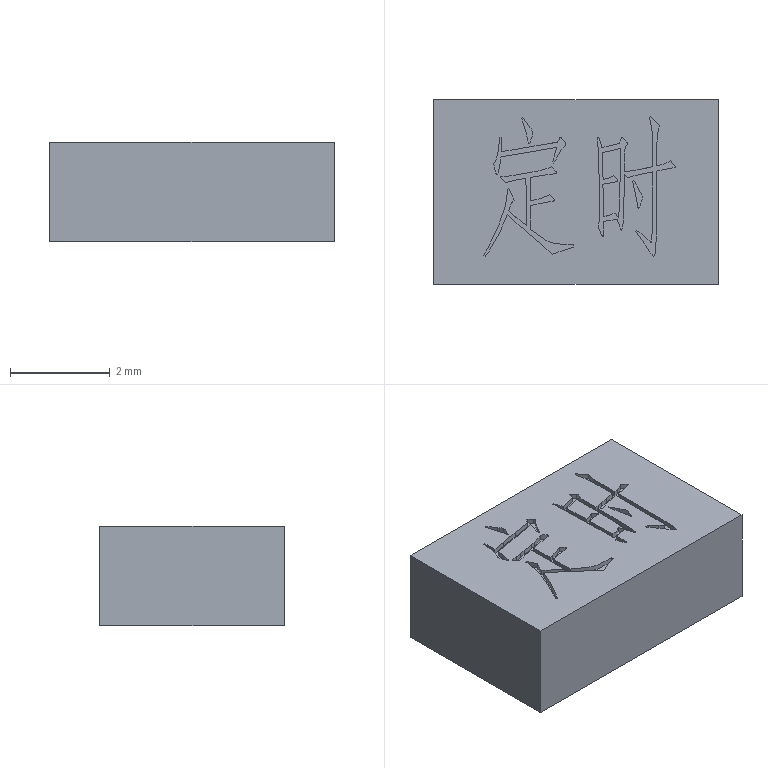Component | SolidWorks | Button3-1 | 1 solid | 162 faces | box 5.7 x 3.7 x 2 mm | volume 42 mm3 | plane 117 | spline 45
build123d program:
from build123d import *

# Parameters (mm, degrees)
SKETCH1_W           = 5.7
SKETCH1_H           = 3.7
BOSS_EXTRUDE1_DEPTH = 2
CUT_EXTRUDE1_DEPTH  = 0.1


with BuildPart() as part:
    # Sketch1 → Boss-Extrude1 (new body)
    with BuildSketch(Plane.XY):
        with Locations((2.85, 1.85)):
            Rectangle(SKETCH1_W, SKETCH1_H)
    extrude(amount=BOSS_EXTRUDE1_DEPTH)

    # Sketch2 → Cut-Extrude1 (cut)
    # profile 1 of 5: a face of its own
    with BuildSketch(Plane.XY.offset(2)):
        with BuildLine():
            Line((1.002, 0.5857), (1.037, 0.6457))
            add(Edge.make_bspline(
                [(1.037, 0.6457), (1.038, 0.6476), (1.041, 0.6531), (1.047, 0.6641), (1.055, 0.6808), (1.062, 0.6935), (1.066, 0.7007)],
                knots=[0, 0, 0, 0, 0.405, 1.215, 2.417, 4, 4, 4, 4], degree=3))
            Line((1.066, 0.7007), (1.146, 0.8473))
            add(Edge.make_bspline(
                [(1.146, 0.8473), (1.16, 0.8735), (1.189, 0.9291), (1.23, 1.019), (1.275, 1.121), (1.313, 1.211), (1.343, 1.286), (1.364, 1.341), (1.383, 1.393), (1.399, 1.442), (1.413, 1.488), (1.426, 1.531), (1.436, 1.572), (1.452, 1.647), (1.468, 1.758), (1.476, 1.856), (1.48, 1.906)],
                knots=[0, 0, 0, 0, 1.106, 2.349, 3.736, 5.256, 6.032, 6.768, 7.459, 8.107, 8.709, 9.274, 9.795, 10.281, 12.137, 14, 14, 14, 14], degree=3))
            Line((1.48, 1.906), (1.506, 1.911))
            Line((1.506, 1.911), (1.609, 1.687))
            add(Edge.make_bspline(
                [(1.609, 1.687), (1.601, 1.681), (1.587, 1.669), (1.573, 1.652), (1.566, 1.638), (1.561, 1.627), (1.554, 1.611), (1.547, 1.591), (1.537, 1.567), (1.528, 1.538), (1.515, 1.505), (1.507, 1.481), (1.503, 1.469)],
                knots=[0, 0, 0, 0, 1.223, 2.28, 2.612, 3.122, 3.811, 4.68, 5.735, 6.98, 8.395, 10, 10, 10, 10], degree=3))
            add(Edge.make_bspline(
                [(1.503, 1.469), (1.527, 1.447), (1.578, 1.401), (1.661, 1.331), (1.754, 1.255), (1.819, 1.202), (1.854, 1.175)],
                knots=[0, 0, 0, 0, 0.8497, 1.799, 2.85, 4, 4, 4, 4], degree=3))
            Line((1.854, 1.175), (1.848, 2.122))
            add(Edge.make_bspline(
                [(1.848, 2.122), (1.814, 2.116), (1.744, 2.106), (1.642, 2.086), (1.541, 2.062), (1.475, 2.042), (1.443, 2.032)],
                knots=[0, 0, 0, 0, 1.012, 2.016, 3.011, 4, 4, 4, 4], degree=3))
            Line((1.443, 2.032), (1.356, 2.122))
            add(Edge.make_bspline(
                [(1.356, 2.122), (1.352, 2.126), (1.344, 2.133), (1.339, 2.148), (1.35, 2.158), (1.359, 2.159), (1.365, 2.159)],
                knots=[0, 0, 0, 0, 1.34, 2.141, 2.818, 4, 4, 4, 4], degree=3))
            Line((1.365, 2.159), (1.474, 2.165))
            Line((1.474, 2.165), (1.612, 2.182))
            Line((1.612, 2.182), (1.739, 2.205))
            Line((1.739, 2.205), (1.989, 2.251))
            Line((1.989, 2.251), (2.084, 2.268))
            add(Edge.make_bspline(
                [(2.084, 2.268), (2.112, 2.274), (2.164, 2.284), (2.236, 2.305), (2.299, 2.328), (2.335, 2.348), (2.352, 2.358)],
                knots=[0, 0, 0, 0, 1.191, 2.249, 3.183, 4, 4, 4, 4], degree=3))
            Line((2.352, 2.358), (2.449, 2.266))
            add(Edge.make_bspline(
                [(2.449, 2.266), (2.454, 2.26), (2.462, 2.25), (2.466, 2.232), (2.455, 2.219), (2.444, 2.218), (2.438, 2.217)],
                knots=[0, 0, 0, 0, 1.282, 2.156, 2.913, 4, 4, 4, 4], degree=3))
            Line((2.438, 2.217), (2.225, 2.188))
            Line((2.225, 2.188), (1.934, 2.139))
            Line((1.934, 2.139), (1.94, 1.67))
            Line((1.94, 1.67), (2.026, 1.69))
            add(Edge.make_bspline(
                [(2.026, 1.69), (2.056, 1.697), (2.113, 1.711), (2.191, 1.736), (2.259, 1.762), (2.299, 1.784), (2.317, 1.794)],
                knots=[0, 0, 0, 0, 1.192, 2.254, 3.188, 4, 4, 4, 4], degree=3))
            Line((2.317, 1.794), (2.406, 1.713))
            add(Edge.make_bspline(
                [(2.406, 1.713), (2.41, 1.709), (2.417, 1.701), (2.42, 1.684), (2.409, 1.67), (2.398, 1.668), (2.392, 1.667)],
                knots=[0, 0, 0, 0, 1.09, 1.984, 2.849, 4, 4, 4, 4], degree=3))
            Line((2.392, 1.667), (2.196, 1.63))
            Line((2.196, 1.63), (1.94, 1.578))
            Line((1.94, 1.578), (1.94, 1.1))
            add(Edge.make_bspline(
                [(1.94, 1.1), (1.964, 1.082), (2.009, 1.047), (2.074, 0.9987), (2.135, 0.9562), (2.19, 0.9196), (2.24, 0.8891), (2.285, 0.8642), (2.324, 0.8455), (2.361, 0.8323), (2.398, 0.823), (2.439, 0.8163), (2.484, 0.809), (2.536, 0.8045), (2.594, 0.7998), (2.657, 0.7979), (2.725, 0.7952), (2.773, 0.7953), (2.797, 0.7953)],
                knots=[0, 0, 0, 0, 1.521, 2.911, 4.161, 5.292, 6.285, 7.162, 7.906, 8.53, 9.144, 9.844, 10.637, 11.519, 12.501, 13.569, 14.737, 16, 16, 16, 16], degree=3))
            Line((2.797, 0.7953), (2.8, 0.7438))
            Line((2.8, 0.7438), (2.53, 0.6572))
            Line((2.53, 0.6572), (2.378, 0.5997))
            add(Edge.make_bspline(
                [(2.378, 0.5997), (2.357, 0.6182), (2.319, 0.6526), (2.265, 0.7007), (2.221, 0.7419), (2.194, 0.767), (2.182, 0.7783)],
                knots=[0, 0, 0, 0, 1.253, 2.338, 3.258, 4, 4, 4, 4], degree=3))
            Line((2.182, 0.7783), (1.796, 1.109))
            Line((1.796, 1.109), (1.477, 1.397))
            add(Edge.make_bspline(
                [(1.477, 1.397), (1.468, 1.374), (1.45, 1.332), (1.425, 1.27), (1.401, 1.213), (1.378, 1.161), (1.357, 1.114), (1.337, 1.071), (1.319, 1.034), (1.297, 0.9906), (1.271, 0.9417), (1.241, 0.8865), (1.211, 0.8345), (1.183, 0.787), (1.159, 0.7452), (1.137, 0.7116), (1.122, 0.6859), (1.113, 0.6719), (1.109, 0.6662)],
                knots=[0, 0, 0, 0, 1.403, 2.709, 3.92, 5.027, 6.04, 6.949, 7.764, 8.482, 9.781, 11.006, 12.172, 13.273, 14.243, 15.016, 15.603, 16, 16, 16, 16], degree=3))
            Line((1.109, 0.6662), (1.071, 0.6172))
            Line((1.071, 0.6172), (1.028, 0.5511))
            Line((1.028, 0.5511), (1.002, 0.5857))
        make_face()
    # profile 2 of 5: a face of its own
    with BuildSketch(Plane.XY.offset(2)):
        with BuildLine():
            Line((1.362, 2.657), (1.655, 2.705))
            Line((1.655, 2.705), (2.049, 2.774))
            Line((2.049, 2.774), (2.475, 2.846))
            Line((2.475, 2.846), (2.521, 2.927))
            add(Edge.make_bspline(
                [(2.521, 2.927), (2.524, 2.932), (2.529, 2.939), (2.535, 2.949), (2.542, 2.947), (2.547, 2.942), (2.555, 2.934), (2.561, 2.928), (2.564, 2.924)],
                knots=[0, 0, 0, 0, 1.715, 2.51, 2.842, 3.5, 4.579, 6, 6, 6, 6], degree=3))
            Line((2.564, 2.924), (2.636, 2.838))
            add(Edge.make_bspline(
                [(2.636, 2.838), (2.64, 2.832), (2.647, 2.822), (2.65, 2.805), (2.646, 2.791), (2.64, 2.784), (2.636, 2.78)],
                knots=[0, 0, 0, 0, 1.322, 2.262, 3.07, 4, 4, 4, 4], degree=3))
            Line((2.636, 2.78), (2.61, 2.76))
            add(Edge.make_bspline(
                [(2.61, 2.76), (2.602, 2.752), (2.584, 2.733), (2.559, 2.696), (2.529, 2.65), (2.509, 2.615), (2.498, 2.596)],
                knots=[0, 0, 0, 0, 0.6907, 1.584, 2.685, 4, 4, 4, 4], degree=3))
            Line((2.498, 2.596), (2.426, 2.464))
            Line((2.426, 2.464), (2.406, 2.427))
            Line((2.406, 2.427), (2.383, 2.45))
            Line((2.383, 2.45), (2.398, 2.507))
            Line((2.398, 2.507), (2.467, 2.743))
            Line((2.467, 2.743), (1.923, 2.648))
            Line((1.923, 2.648), (1.35, 2.553))
            add(Edge.make_bspline(
                [(1.35, 2.553), (1.348, 2.536), (1.344, 2.504), (1.338, 2.46), (1.334, 2.424), (1.329, 2.394), (1.324, 2.364), (1.316, 2.331), (1.307, 2.291), (1.298, 2.255), (1.29, 2.226), (1.284, 2.21), (1.278, 2.198), (1.272, 2.191), (1.263, 2.191), (1.257, 2.198), (1.252, 2.21), (1.249, 2.22), (1.247, 2.225)],
                knots=[0, 0, 0, 0, 2.01, 3.724, 5.107, 6.182, 7.226, 8.53, 10.107, 11.945, 12.829, 13.511, 13.979, 14.291, 14.536, 14.848, 15.323, 16, 16, 16, 16], degree=3))
            Line((1.247, 2.225), (1.224, 2.3))
            Line((1.224, 2.3), (1.209, 2.369))
            add(Edge.make_bspline(
                [(1.209, 2.369), (1.207, 2.378), (1.204, 2.394), (1.204, 2.414), (1.209, 2.427), (1.215, 2.439), (1.224, 2.453), (1.237, 2.471), (1.25, 2.497), (1.263, 2.533), (1.274, 2.58), (1.286, 2.635), (1.296, 2.693), (1.305, 2.749), (1.31, 2.801), (1.312, 2.834), (1.313, 2.849)],
                knots=[0, 0, 0, 0, 0.79, 1.34, 1.62, 2, 2.477, 3.064, 3.834, 4.889, 6.248, 7.899, 9.634, 11.229, 12.683, 14, 14, 14, 14], degree=3))
            Line((1.313, 2.849), (1.316, 2.942))
            Line((1.316, 2.942), (1.35, 2.944))
            Line((1.35, 2.944), (1.356, 2.869))
            add(Edge.make_bspline(
                [(1.356, 2.869), (1.357, 2.849), (1.359, 2.809), (1.361, 2.768), (1.362, 2.749)],
                knots=[0, 0, 0, 0, 1.025, 2, 2, 2, 2], degree=3))
            Line((1.362, 2.749), (1.362, 2.657))
        make_face()
    # profile 3 of 5: a face of its own
    with BuildSketch(Plane.XY.offset(2)):
        with BuildLine():
            Line((1.762, 3.321), (1.788, 3.347))
            Line((1.788, 3.347), (1.814, 3.307))
            Line((1.814, 3.307), (1.929, 3.146))
            Line((1.929, 3.146), (1.952, 3.114))
            add(Edge.make_bspline(
                [(1.952, 3.114), (1.957, 3.105), (1.967, 3.09), (1.979, 3.068), (1.986, 3.052), (1.989, 3.035), (1.985, 3.015), (1.982, 2.999), (1.98, 2.991)],
                knots=[0, 0, 0, 0, 1.399, 2.492, 3.295, 3.839, 4.808, 6, 6, 6, 6], degree=3))
            Line((1.98, 2.991), (1.957, 2.918))
            Line((1.957, 2.918), (1.94, 2.866))
            add(Edge.make_bspline(
                [(1.94, 2.866), (1.938, 2.86), (1.933, 2.847), (1.925, 2.831), (1.919, 2.82), (1.912, 2.813), (1.904, 2.814), (1.899, 2.821), (1.894, 2.832), (1.892, 2.841), (1.891, 2.846)],
                knots=[0, 0, 0, 0, 1.762, 3.131, 4.119, 4.759, 5.226, 5.791, 6.7, 8, 8, 8, 8], degree=3))
            Line((1.891, 2.846), (1.883, 2.884))
            Line((1.883, 2.884), (1.862, 2.991))
            add(Edge.make_bspline(
                [(1.862, 2.991), (1.858, 3.009), (1.848, 3.05), (1.829, 3.115), (1.806, 3.189), (1.789, 3.242), (1.779, 3.269)],
                knots=[0, 0, 0, 0, 0.7957, 1.728, 2.796, 4, 4, 4, 4], degree=3))
            Line((1.779, 3.269), (1.762, 3.321))
        make_face()
    # profile 4 of 5: a face of its own
    with BuildSketch(Plane.XY.offset(2)):
        with BuildLine():
            Line((3.308, 2.939), (3.369, 2.734))
            Line((3.369, 2.734), (3.717, 2.823))
            Line((3.717, 2.823), (3.751, 2.916))
            add(Edge.make_bspline(
                [(3.751, 2.916), (3.753, 2.921), (3.755, 2.93), (3.764, 2.942), (3.779, 2.935), (3.787, 2.928), (3.792, 2.924)],
                knots=[0, 0, 0, 0, 1.235, 1.874, 2.609, 4, 4, 4, 4], degree=3))
            Line((3.792, 2.924), (3.861, 2.846))
            add(Edge.make_bspline(
                [(3.861, 2.846), (3.865, 2.841), (3.872, 2.832), (3.878, 2.815), (3.869, 2.798), (3.854, 2.777), (3.838, 2.744), (3.829, 2.71), (3.824, 2.675), (3.822, 2.641), (3.82, 2.601), (3.82, 2.572), (3.82, 2.556)],
                knots=[0, 0, 0, 0, 0.6995, 1.132, 1.626, 2.527, 3.71, 5.139, 6.026, 7.129, 8.454, 10, 10, 10, 10], degree=3))
            Line((3.82, 2.556), (3.818, 2.257))
            Line((3.818, 2.257), (3.887, 2.263))
            Line((3.887, 2.263), (4.01, 2.28))
            Line((4.01, 2.28), (4.174, 2.312))
            Line((4.174, 2.312), (4.384, 2.355))
            Line((4.384, 2.355), (4.384, 2.936))
            add(Edge.make_bspline(
                [(4.384, 2.936), (4.384, 2.944), (4.384, 2.963), (4.382, 2.992), (4.379, 3.025), (4.374, 3.071), (4.367, 3.126), (4.359, 3.18), (4.351, 3.222), (4.342, 3.258), (4.331, 3.298), (4.322, 3.326), (4.318, 3.341)],
                knots=[0, 0, 0, 0, 0.6304, 1.345, 2.132, 3.005, 4.724, 6.211, 6.969, 7.851, 8.859, 10, 10, 10, 10], degree=3))
            Line((4.318, 3.341), (4.341, 3.364))
            Line((4.341, 3.364), (4.519, 3.172))
            add(Edge.make_bspline(
                [(4.519, 3.172), (4.514, 3.154), (4.503, 3.122), (4.49, 3.074), (4.481, 3.03), (4.474, 2.976), (4.471, 2.907), (4.471, 2.852), (4.47, 2.823)],
                knots=[0, 0, 0, 0, 0.9187, 1.75, 2.509, 3.194, 4.54, 6, 6, 6, 6], degree=3))
            Line((4.47, 2.823), (4.467, 2.369))
            Line((4.467, 2.369), (4.568, 2.395))
            add(Edge.make_bspline(
                [(4.568, 2.395), (4.584, 2.399), (4.615, 2.407), (4.659, 2.425), (4.699, 2.446), (4.723, 2.464), (4.735, 2.473)],
                knots=[0, 0, 0, 0, 1.06, 2.069, 3.045, 4, 4, 4, 4], degree=3))
            Line((4.735, 2.473), (4.827, 2.378))
            add(Edge.make_bspline(
                [(4.827, 2.378), (4.83, 2.373), (4.836, 2.365), (4.84, 2.353), (4.836, 2.341), (4.828, 2.34), (4.824, 2.34)],
                knots=[0, 0, 0, 0, 1.301, 2.329, 3.072, 4, 4, 4, 4], degree=3))
            Line((4.824, 2.34), (4.787, 2.332))
            add(Edge.make_bspline(
                [(4.787, 2.332), (4.785, 2.331), (4.779, 2.329), (4.766, 2.327), (4.746, 2.323), (4.724, 2.321), (4.701, 2.318), (4.68, 2.314), (4.654, 2.308), (4.624, 2.303), (4.591, 2.295), (4.553, 2.288), (4.512, 2.278), (4.483, 2.272), (4.467, 2.268)],
                knots=[0, 0, 0, 0, 0.1987, 0.6791, 1.428, 2.474, 3.14, 3.954, 4.915, 6.017, 7.286, 8.716, 10.278, 12, 12, 12, 12], degree=3))
            Line((4.467, 2.268), (4.462, 1.028))
            add(Edge.make_bspline(
                [(4.462, 1.028), (4.462, 1.027), (4.461, 1.024), (4.461, 1.016), (4.46, 1.004), (4.459, 0.9887), (4.458, 0.9688), (4.458, 0.9448), (4.457, 0.9168), (4.456, 0.8749), (4.454, 0.8223), (4.451, 0.7623), (4.447, 0.7078), (4.441, 0.66), (4.435, 0.6201), (4.426, 0.5908), (4.419, 0.5716), (4.407, 0.5624), (4.397, 0.5658), (4.389, 0.5712), (4.379, 0.5799), (4.368, 0.5924), (4.356, 0.6089), (4.341, 0.6283), (4.326, 0.6518), (4.315, 0.6687), (4.309, 0.6777)],
                knots=[0, 0, 0, 0, 0.1346, 0.4289, 0.8709, 1.476, 2.244, 3.158, 4.236, 5.461, 7.976, 10.282, 12.361, 14.252, 15.825, 16.982, 17.742, 18.232, 18.485, 18.852, 19.35, 19.985, 20.766, 21.7, 22.782, 24, 24, 24, 24], degree=3))
            Line((4.309, 0.6777), (4.209, 0.8298))
            Line((4.209, 0.8298), (4.088, 0.9909))
            Line((4.088, 0.9909), (4.045, 1.051))
            Line((4.045, 1.051), (4.059, 1.086))
            Line((4.059, 1.086), (4.108, 1.048))
            Line((4.108, 1.048), (4.266, 0.9164))
            add(Edge.make_bspline(
                [(4.266, 0.9164), (4.279, 0.906), (4.3, 0.888), (4.328, 0.8632), (4.346, 0.8519), (4.359, 0.8396), (4.367, 0.8508), (4.367, 0.8676), (4.37, 0.8955), (4.37, 0.9178), (4.37, 0.9308)],
                knots=[0, 0, 0, 0, 1.858, 3.233, 4.127, 4.549, 4.814, 5.443, 6.503, 8, 8, 8, 8], degree=3))
            Line((4.37, 0.9308), (4.375, 1.141))
            Line((4.375, 1.141), (4.384, 2.251))
            add(Edge.make_bspline(
                [(4.384, 2.251), (4.343, 2.244), (4.26, 2.231), (4.135, 2.205), (4.011, 2.173), (3.928, 2.148), (3.887, 2.136)],
                knots=[0, 0, 0, 0, 0.9818, 1.977, 2.982, 4, 4, 4, 4], degree=3))
            Line((3.887, 2.136), (3.818, 2.205))
            Line((3.818, 2.205), (3.809, 1.584))
            add(Edge.make_bspline(
                [(3.809, 1.584), (3.808, 1.561), (3.806, 1.512), (3.803, 1.45), (3.802, 1.398), (3.8, 1.364), (3.799, 1.335), (3.798, 1.318), (3.797, 1.311)],
                knots=[0, 0, 0, 0, 1.469, 3.229, 4.108, 4.866, 5.494, 6, 6, 6, 6], degree=3))
            Line((3.797, 1.311), (3.792, 1.219))
            add(Edge.make_bspline(
                [(3.792, 1.219), (3.791, 1.21), (3.789, 1.195), (3.787, 1.174), (3.785, 1.159), (3.782, 1.143), (3.776, 1.122), (3.769, 1.103), (3.763, 1.09), (3.758, 1.087), (3.752, 1.089), (3.748, 1.095), (3.742, 1.104), (3.737, 1.118), (3.732, 1.135), (3.728, 1.148), (3.726, 1.155)],
                knots=[0, 0, 0, 0, 1.645, 2.981, 4.015, 4.743, 6.147, 8.198, 8.682, 8.992, 9.281, 9.752, 10.46, 11.39, 12.581, 14, 14, 14, 14], degree=3))
            Line((3.726, 1.155), (3.677, 1.305))
            Line((3.677, 1.305), (3.403, 1.259))
            Line((3.403, 1.259), (3.4, 1.066))
            add(Edge.make_bspline(
                [(3.4, 1.066), (3.4, 1.052), (3.399, 1.029), (3.397, 0.9987), (3.395, 0.9787), (3.392, 0.9676), (3.388, 0.9611), (3.384, 0.962), (3.383, 0.9624)],
                knots=[0, 0, 0, 0, 2.223, 3.847, 4.918, 5.43, 5.79, 6, 6, 6, 6], degree=3))
            add(Edge.make_bspline(
                [(3.383, 0.9624), (3.38, 0.9629), (3.375, 0.964), (3.369, 0.9712), (3.362, 0.981), (3.359, 0.9893), (3.357, 0.9939)],
                knots=[0, 0, 0, 0, 0.6727, 1.496, 2.598, 4, 4, 4, 4], degree=3))
            Line((3.357, 0.9939), (3.317, 1.094))
            add(Edge.make_bspline(
                [(3.317, 1.094), (3.313, 1.105), (3.305, 1.124), (3.296, 1.149), (3.291, 1.169), (3.291, 1.18), (3.291, 1.184)],
                knots=[0, 0, 0, 0, 1.446, 2.596, 3.435, 4, 4, 4, 4], degree=3))
            add(Edge.make_bspline(
                [(3.291, 1.184), (3.291, 1.186), (3.292, 1.19), (3.294, 1.198), (3.297, 1.21), (3.305, 1.231), (3.313, 1.265), (3.317, 1.31), (3.32, 1.36), (3.321, 1.401), (3.322, 1.432), (3.322, 1.45), (3.323, 1.463), (3.323, 1.469), (3.323, 1.472)],
                knots=[0, 0, 0, 0, 0.1966, 0.542, 1.054, 1.721, 3.35, 5.278, 7.373, 9.485, 10.452, 11.191, 11.701, 12, 12, 12, 12], degree=3))
            Line((3.323, 1.472), (3.314, 2.093))
            Line((3.314, 2.093), (3.297, 2.654))
            Line((3.297, 2.654), (3.279, 2.933))
            Line((3.279, 2.933), (3.308, 2.939))
        make_face()
        with BuildLine():
            add(Edge.make_bspline(
                [(3.392, 2.102), (3.413, 2.105), (3.455, 2.112), (3.513, 2.128), (3.565, 2.148), (3.596, 2.165), (3.61, 2.174)],
                knots=[0, 0, 0, 0, 1.13, 2.169, 3.118, 4, 4, 4, 4], degree=3))
            Line((3.61, 2.174), (3.679, 2.093))
            add(Edge.make_bspline(
                [(3.679, 2.093), (3.683, 2.089), (3.688, 2.081), (3.691, 2.068), (3.684, 2.055), (3.676, 2.053), (3.671, 2.053)],
                knots=[0, 0, 0, 0, 1.184, 2.115, 2.913, 4, 4, 4, 4], degree=3))
            Line((3.671, 2.053), (3.389, 2.004))
            Line((3.389, 2.004), (3.403, 1.357))
            add(Edge.make_bspline(
                [(3.403, 1.357), (3.417, 1.36), (3.444, 1.366), (3.482, 1.374), (3.517, 1.384), (3.548, 1.392), (3.575, 1.4), (3.599, 1.409), (3.619, 1.417), (3.631, 1.423), (3.636, 1.426)],
                knots=[0, 0, 0, 0, 1.407, 2.702, 3.875, 4.935, 5.874, 6.694, 7.405, 8, 8, 8, 8], degree=3))
            Line((3.636, 1.426), (3.7, 1.342))
            add(Edge.make_bspline(
                [(3.7, 1.342), (3.702, 1.353), (3.706, 1.373), (3.71, 1.4), (3.714, 1.418), (3.715, 1.432), (3.716, 1.446), (3.718, 1.463), (3.719, 1.487), (3.721, 1.515), (3.723, 1.544), (3.724, 1.569), (3.725, 1.59), (3.725, 1.602), (3.726, 1.607)],
                knots=[0, 0, 0, 0, 1.544, 2.753, 3.611, 4.133, 4.634, 5.423, 6.5, 7.847, 9.233, 10.386, 11.309, 12, 12, 12, 12], degree=3))
            Line((3.726, 1.607), (3.74, 2.72))
            Line((3.74, 2.72), (3.377, 2.636))
            Line((3.377, 2.636), (3.392, 2.102))
        make_face(mode=Mode.SUBTRACT)
    # profile 5 of 5: a face of its own
    with BuildSketch(Plane.XY.offset(2)):
        with BuildLine():
            Line((3.984, 2.053), (4.01, 2.081))
            Line((4.01, 2.081), (4.036, 2.035))
            Line((4.036, 2.035), (4.119, 1.877))
            add(Edge.make_bspline(
                [(4.119, 1.877), (4.125, 1.866), (4.135, 1.846), (4.149, 1.819), (4.16, 1.795), (4.17, 1.775), (4.178, 1.759), (4.183, 1.747), (4.186, 1.739), (4.188, 1.732), (4.184, 1.725), (4.182, 1.712), (4.175, 1.694), (4.171, 1.681), (4.168, 1.673)],
                knots=[0, 0, 0, 0, 1.933, 3.61, 5.04, 6.243, 7.179, 7.88, 8.345, 8.58, 8.959, 9.651, 10.669, 12, 12, 12, 12], degree=3))
            Line((4.168, 1.673), (4.134, 1.578))
            add(Edge.make_bspline(
                [(4.134, 1.578), (4.131, 1.571), (4.126, 1.558), (4.116, 1.542), (4.109, 1.532), (4.102, 1.526), (4.094, 1.529), (4.09, 1.536), (4.088, 1.547), (4.088, 1.556), (4.088, 1.561)],
                knots=[0, 0, 0, 0, 1.854, 3.268, 4.259, 4.912, 5.373, 5.938, 6.81, 8, 8, 8, 8], degree=3))
            Line((4.088, 1.561), (4.079, 1.621))
            add(Edge.make_bspline(
                [(4.079, 1.621), (4.078, 1.628), (4.077, 1.644), (4.072, 1.672), (4.066, 1.707), (4.058, 1.746), (4.049, 1.785), (4.043, 1.818), (4.037, 1.844), (4.033, 1.864), (4.029, 1.885), (4.021, 1.911), (4.012, 1.946), (4.006, 1.972), (4.002, 1.986)],
                knots=[0, 0, 0, 0, 0.6757, 1.576, 2.703, 4.072, 5.428, 6.531, 7.372, 7.946, 8.534, 9.41, 10.556, 12, 12, 12, 12], degree=3))
            Line((4.002, 1.986), (3.984, 2.053))
        make_face()
    extrude(amount=-CUT_EXTRUDE1_DEPTH, mode=Mode.SUBTRACT)


solid = part.part

# Placed as in the assembly
solid = solid.moved(Location((-64.106, -4.714, 277.152), (0, 0, 0)))